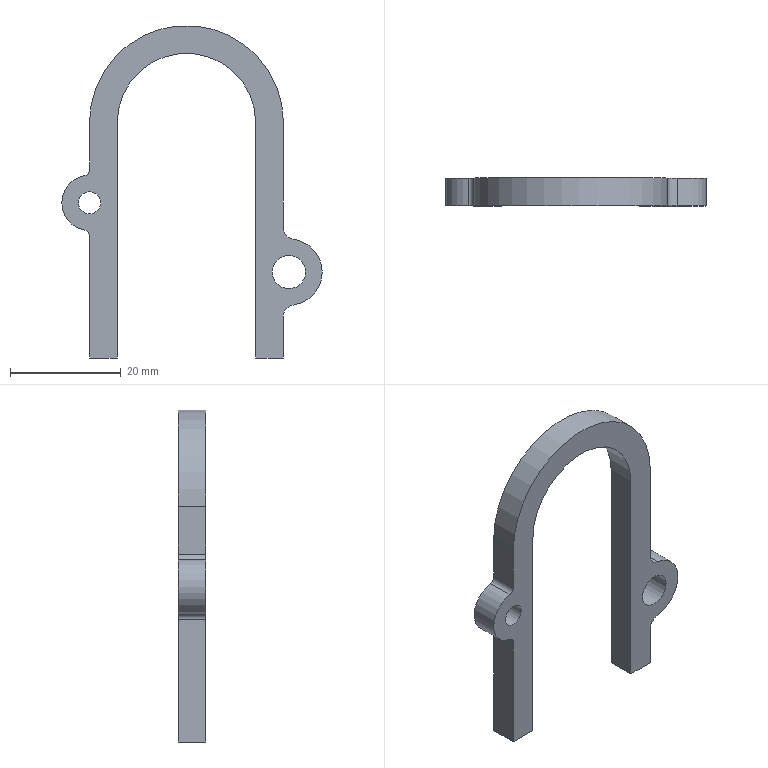Component | NX | RETAINING_RING | 1 solid | 20 faces | volume 3647 mm3 | cylinder 10 | plane 10 | commonest cylinder face diameters 4 x3 2 x2 10 x1 25 x1 12 x1 35 x1 6 x1